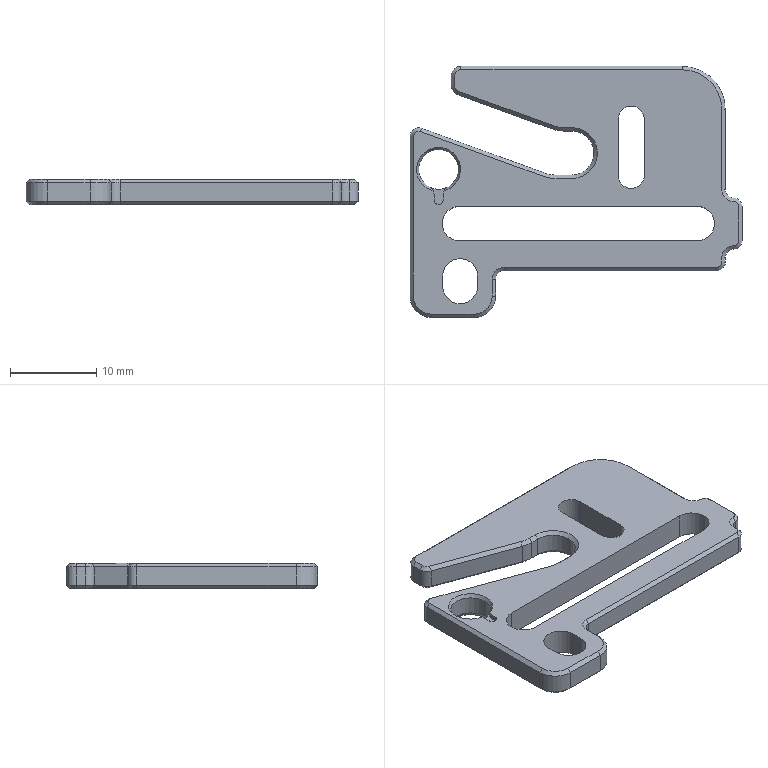CAM job | NX | mm | 3-axis | 4 set-ups | 34 operations | part box 38.6 x 29.21 x 2.99
set-up 1
1. Face Milling | Mill Mill5 T1 | FACE_MILLING | path 433.11 mm | 3.431 min
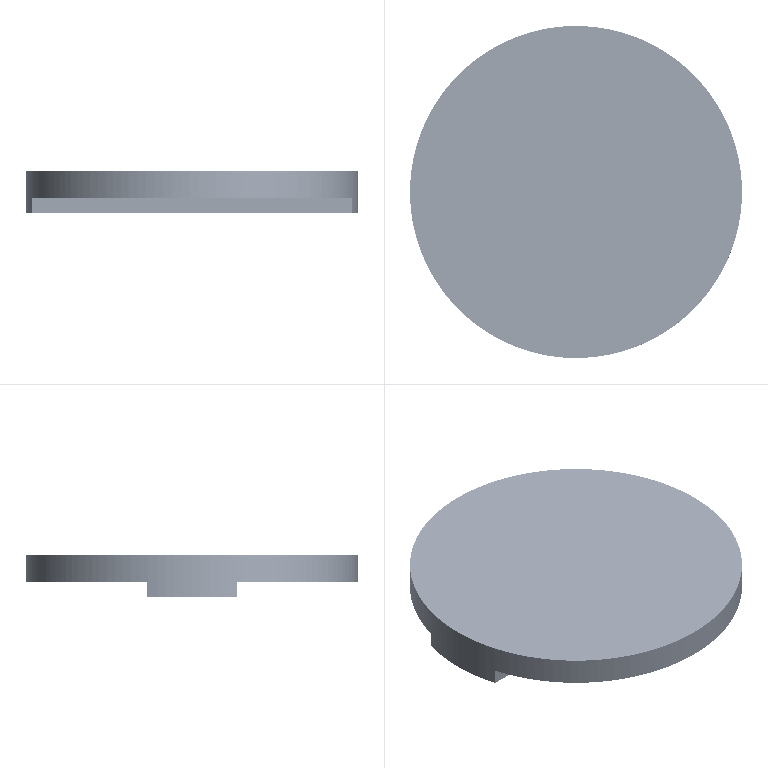2. Planar Milling | Mill Mill5 T09D6C | PLANAR_MILL_COPY | path 187.203 mm | 0.08447 min
set-up 2
3. Cavity Milling | Mill Mill5 T01D10CJG | CAVITY_MILL_1_COPY | path 9793.39 mm | 3.761 min
4. Face Milling | Mill Mill5 T09D6C | FACE_MILLING_COPY | path 318.932 mm | 0.3758 min
5. Planar Milling | Mill Mill5 T09D6C | PLANAR_MILL_COPY_COPY_COPY_COPY_COPY_2 | path 527.949 mm | 0.3661 min
6. Planar Milling | Mill Mill5 T09D6C | PLANAR_MILL_COPY_COPY_COPY_COPY | path 173.211 mm | 0.2119 min
7. Planar Milling | Mill Mill5 T03D3C | PLANAR_MILL_COPY_COPY_COPY_COPY_COPY_2_COPY_1 | path 1552.718 mm | 1.75 min
8. Planar Milling | Mill Mill5 T03D3C | PLANAR_MILL_COPY_COPY_COPY_COPY_COPY_2_COPY_1_COPY | path 1450.505 mm | 1.43 min
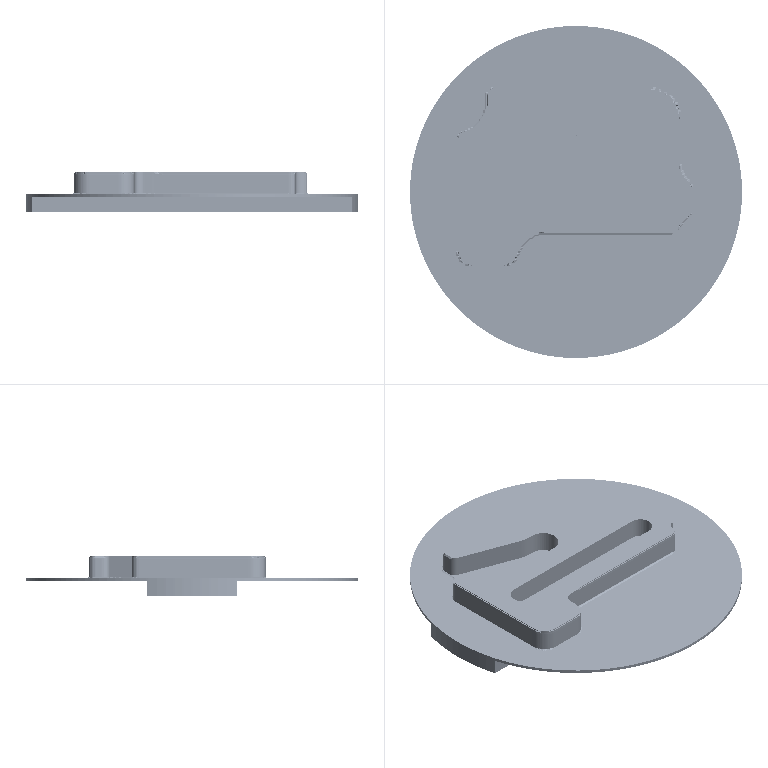9. Planar Milling | Mill Mill5 T03D3C | PLANAR_MILL_COPY_COPY_COPY_COPY_COPY_2_COPY_1_COPY_COPY_1 | path 165.322 mm | 0.1449 min
10. Cylinder Milling | Mill Mill5 T03D3C | HOLE_MILLING_1 | path 141.327 mm | 0.1502 min
11. Planar Milling | Mill Mill5 T07D2.5C | PLANAR_MILL_COPY_COPY_COPY_COPY_COPY_2_COPY_1_COPY_COPY | path 448.236 mm | 0.4278 min
12. Face Milling | Mill Mill5 T02D6J | FACE_MILLING_COPY_COPY_1 | path 319.032 mm | 0.4292 min
13. Planar Milling | Mill Mill5 T02D6J | PLANAR_MILL_COPY_COPY_COPY_COPY_COPY_3 | path 173.041 mm | 0.2465 min
14. Planar Milling | Mill Mill5 T04D2.5J | PLANAR_MILL_COPY_COPY_COPY_COPY_COPY_3_COPY | path 72.169 mm | 0.0796 min
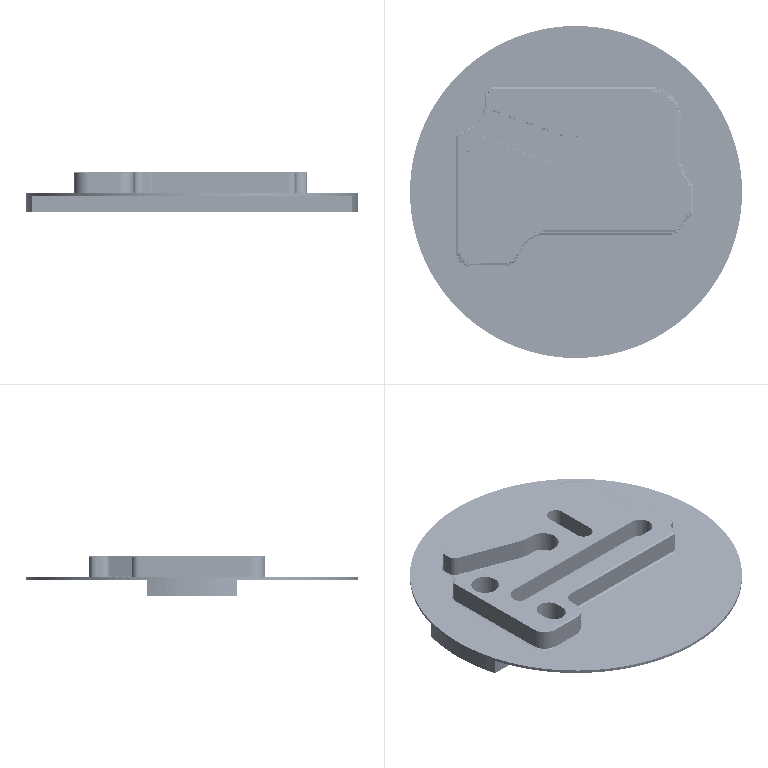15. Planar Milling | Mill Mill5 T04D2.5J | PLANAR_MILL_COPY_COPY_COPY_COPY_COPY_3_COPY_COPY | path 130.367 mm | 0.1499 min
16. Planar Milling | Mill Mill5 T04D2.5J | PLANAR_MILL_COPY_COPY_COPY_COPY_COPY_3_COPY_COPY_COPY | path 42.026 mm | 0.03509 min
17. Planar Milling | Mill Mill5 T04D2.5J | PLANAR_MILL_COPY_COPY_COPY_COPY_COPY_3_COPY_COPY_COPY_1 | path 34.817 mm | 0.02067 min
18. Planar Milling | Mill Mill5 T08D1.5J | PLANAR_MILL_COPY_COPY_COPY_COPY_COPY_3_COPY_1 | path 800.278 mm | 0.7625 min
19. Planar Milling | Mill Mill5 T06D1C | PLANAR_MILL_COPY_COPY_COPY_COPY_COPY_3_COPY_1_COPY | path 155.189 mm | 0.2124 min
20. Planar Milling | Mill Mill5 T06D1C | PLANAR_MILL_COPY_COPY_COPY_COPY_COPY_3_COPY_1_COPY_COPY | path 26.817 mm | 0.02133 min
21. Planar Milling | Mill Mill5 T05D2X90 | PLANAR_MILL_COPY_COPY_COPY_COPY_1_COPY | path 187.991 mm | 0.2104 min
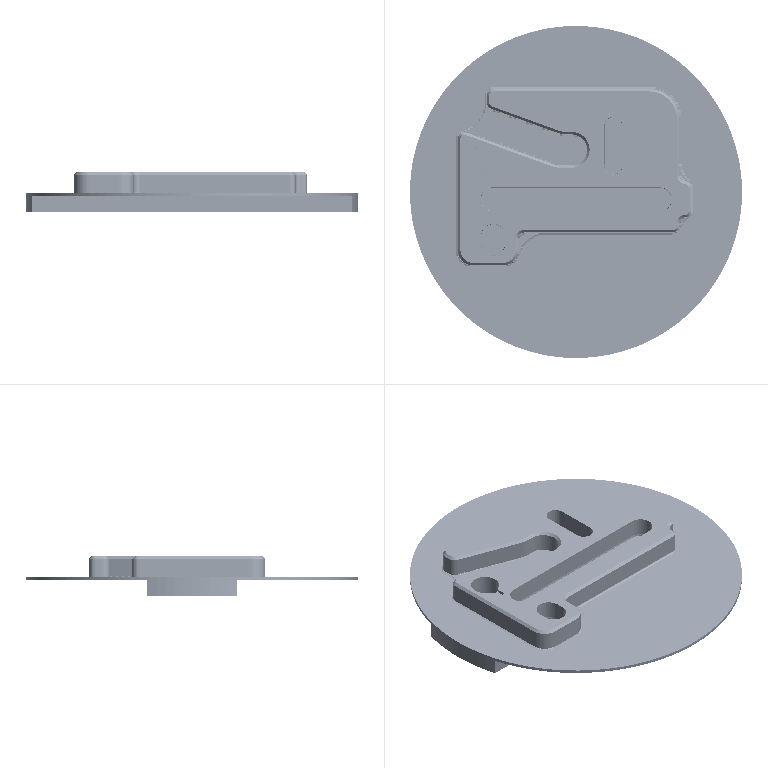22. Planar Milling | Mill Mill5 T05D2X90 | PLANAR_MILL_COPY_COPY_COPY_COPY_1_COPY_COPY | path 238.181 mm | 0.1521 min
23. Planar Milling | Mill Mill5 T05D2X90 | PLANAR_MILL_COPY_COPY_COPY_COPY_1_COPY_COPY_COPY | path 25.601 mm | 0.008311 min
set-up 3
24. Cavity Milling | Mill Mill5 T01D10CJG | CAVITY_MILL_1_COPY_COPY | path 6160.494 mm | 2.777 min
25. Face Milling | Mill Mill5 T02D6J | FACE_MILLING_COPY_COPY_COPY | path 300.395 mm | 0.4693 min
26. Planar Milling | Mill Mill5 T06D1C | PLANAR_MILL_COPY_COPY_COPY_COPY_COPY_3_COPY_1_COPY_COPY_1 | path 155.189 mm | 0.2124 min
27. Planar Milling | Mill Mill5 T06D1C | PLANAR_MILL_COPY_COPY_COPY_COPY_COPY_3_COPY_1_COPY_COPY_COPY | path 26.817 mm | 0.02133 min
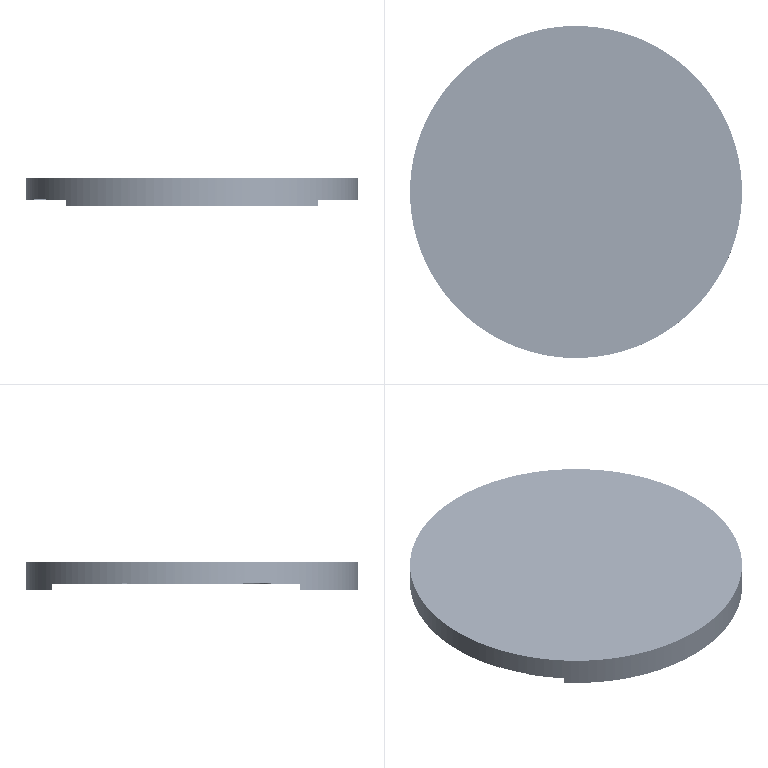28. Planar Milling | Mill Mill5 T05D2X90 | PLANAR_MILL_COPY_COPY_COPY_COPY_1_COPY_COPY_2 | path 187.991 mm | 0.2104 min
29. Planar Milling | Mill Mill5 T05D2X90 | PLANAR_MILL_COPY_COPY_COPY_COPY_1_COPY_COPY_COPY_1 | path 235.656 mm | 0.1518 min
30. Planar Milling | Mill Mill5 T05D2X90 | PLANAR_MILL_COPY_COPY_COPY_COPY_1_COPY_COPY_COPY_COPY | path 27.187 mm | 0.01029 min
set-up 4
31. Cavity Milling | Mill Mill5 T09D6C | CAVITY_MILL | path 1854.944 mm | 1.136 min
32. Cavity Milling | Mill Mill5 T04D2.5J | CAVITY_MILL_COPY | path 622.17 mm | 0.3791 min
33. Cavity Milling | Mill Mill5 T04D2.5J | CAVITY_MILL_COPY_COPY | path 525.899 mm | 0.6278 min
34. Cavity Milling | Mill Mill5 T04D2.5J | CAVITY_MILL_COPY_COPY_COPY | path 152.1 mm | 0.2657 min